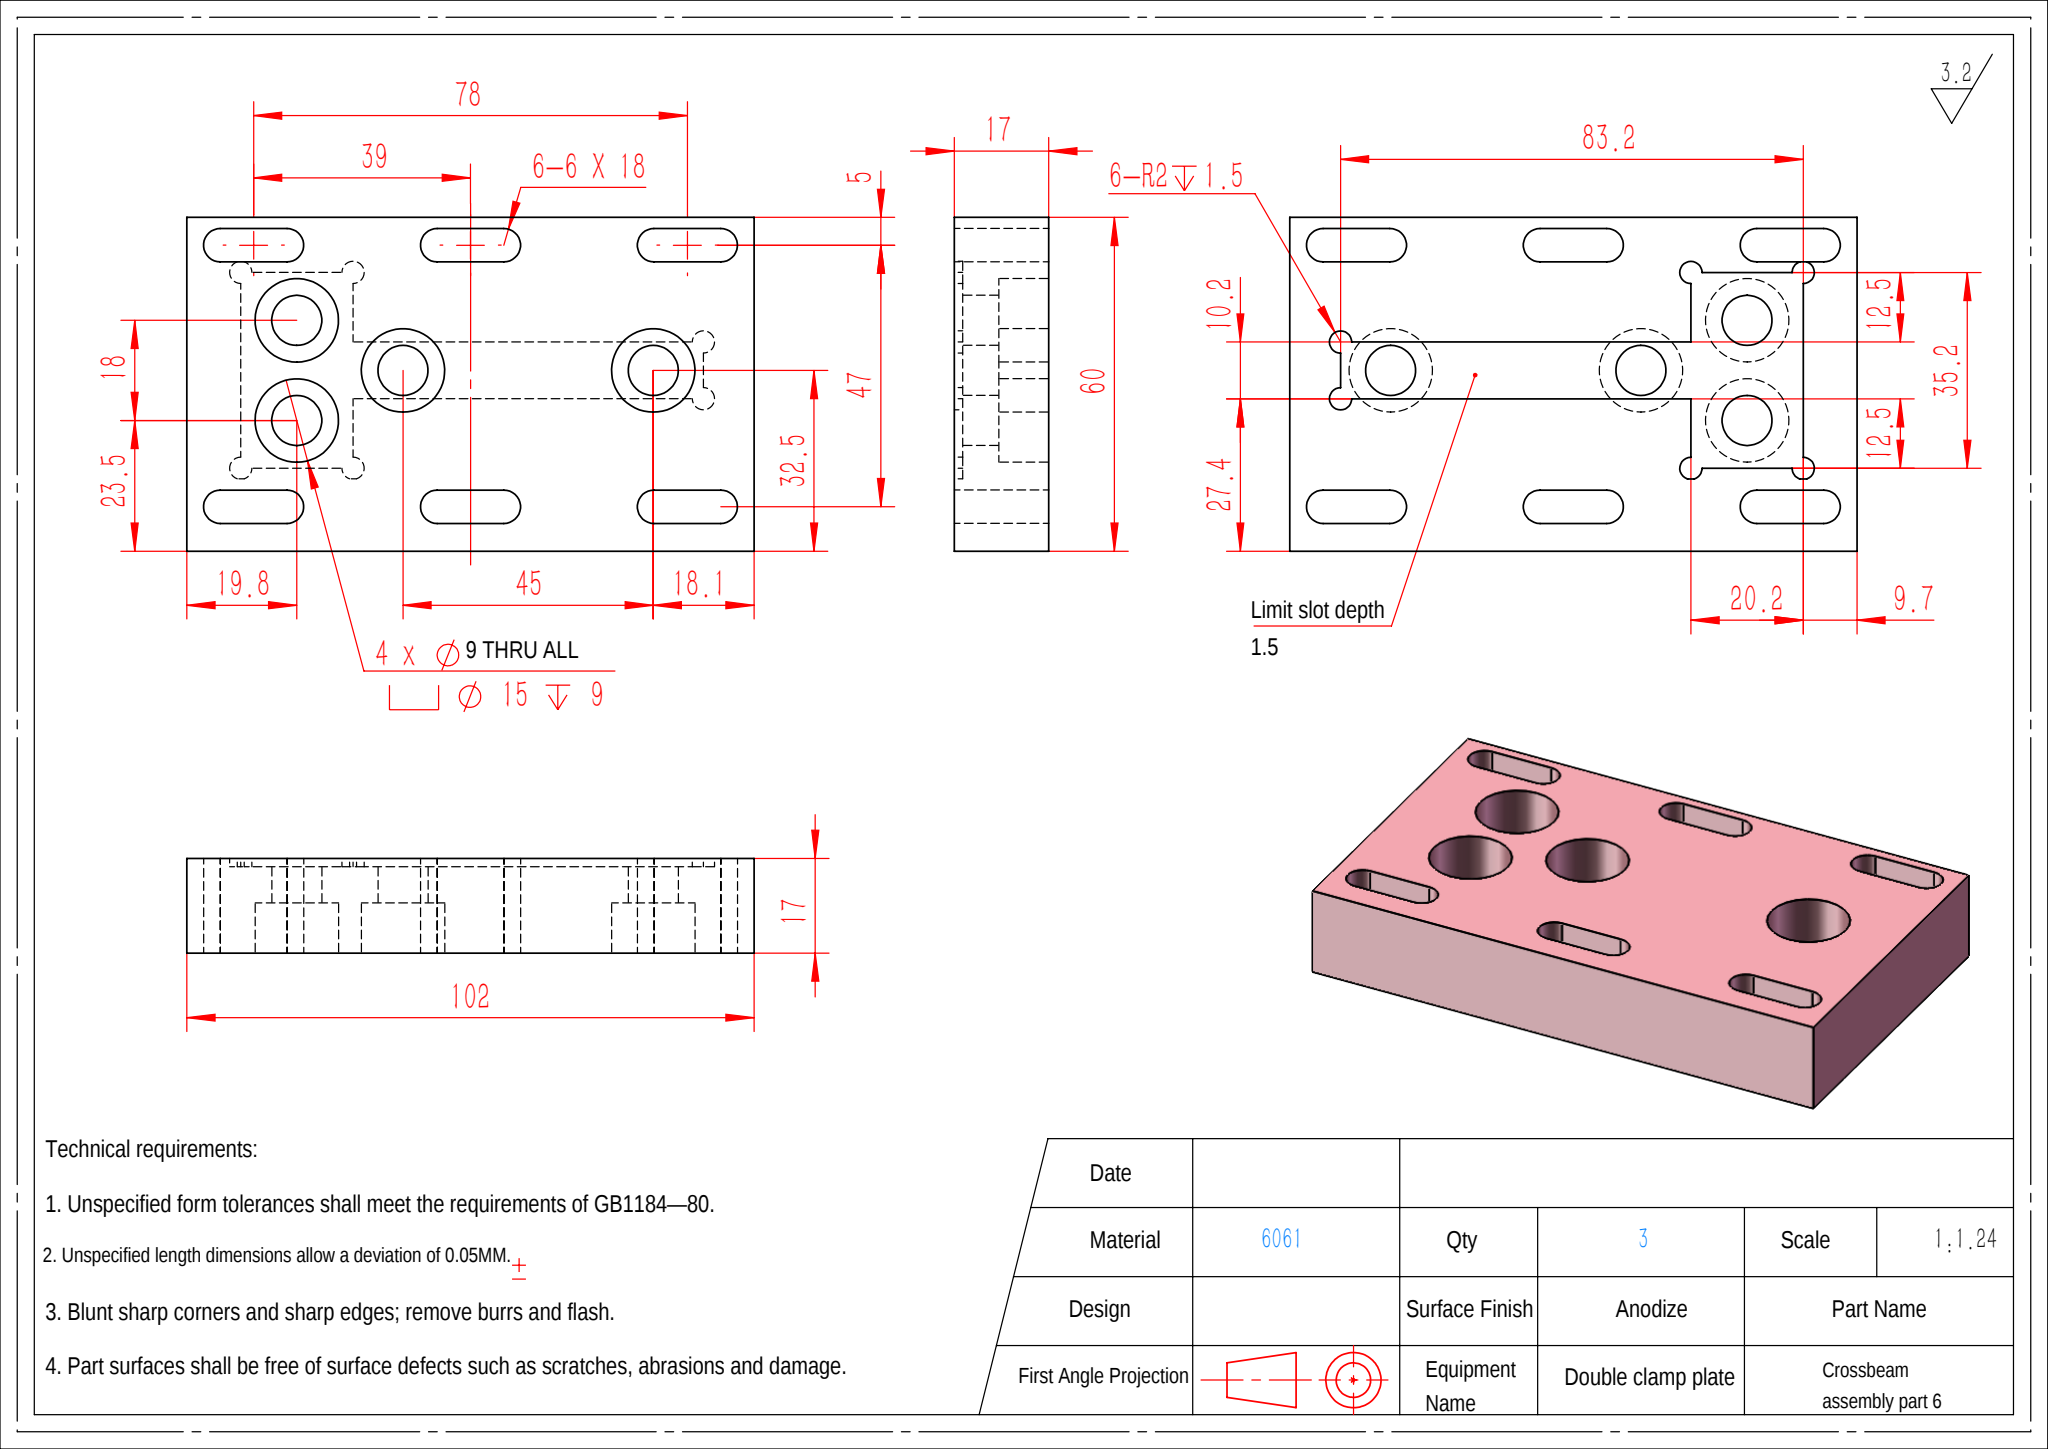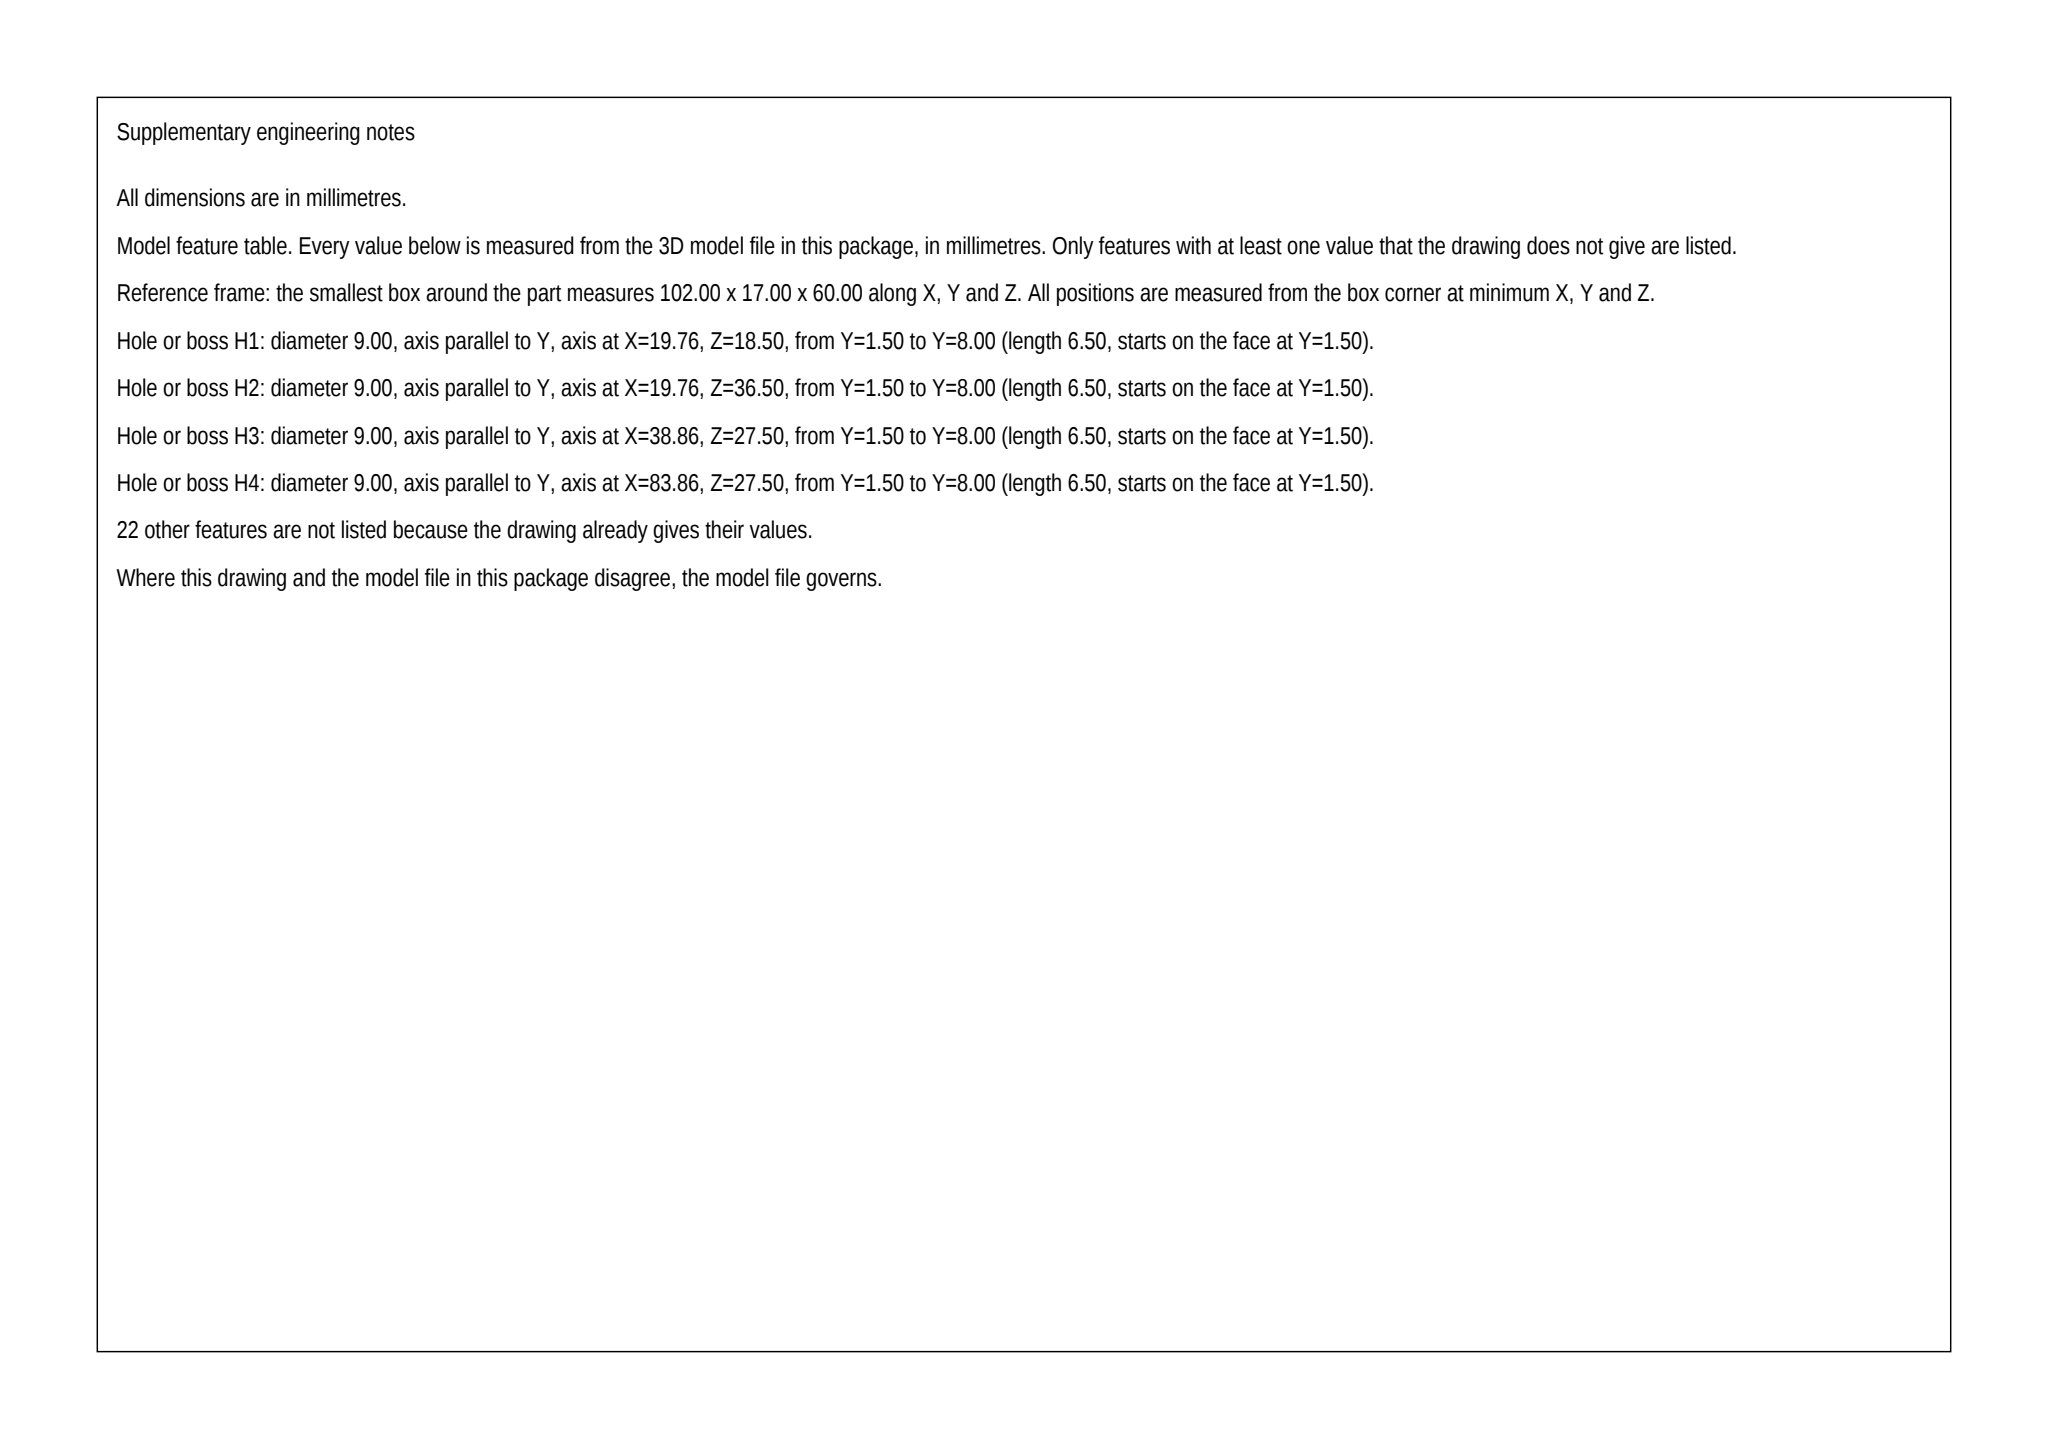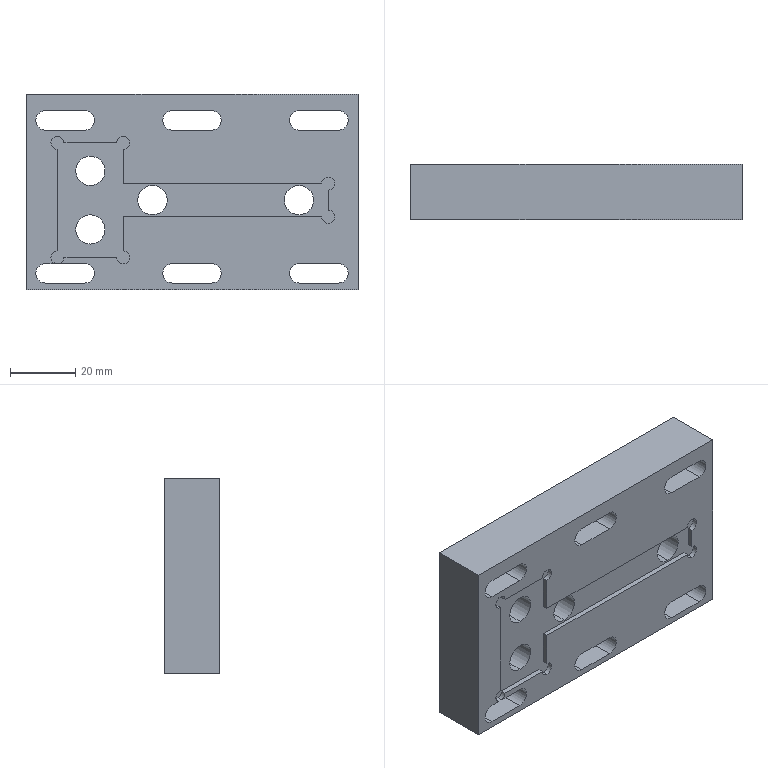Part | SolidWorks | mm | material 6061 | 1 solid | 72 faces | box 102 x 17 x 60 mm | volume 83681 mm3 | cylinder 39 | plane 33 | commonest cylinder face diameters 6 x12 4 x11 15 x8 9 x8
build123d program:
from build123d import *

# Parameters (mm, degrees)
SKETCH1_W                                           = 102
SKETCH1_H                                           = 60
BOSS_EXTRUDE1_DEPTH                                 = 8.5
CUT_EXTRUDE2_DEPTH                                  = 1.5
CUT_EXTRUDE4_DEPTH                                  = 62.563
CYLINDRICAL_COUNTERSUNK_HOLE_FOR_M8_HEX_D           = 9
CYLINDRICAL_COUNTERSUNK_HOLE_FOR_M8_HEX_DEPTH       = 17
CYLINDRICAL_COUNTERSUNK_HOLE_FOR_M8_HEX_CBORE_D     = 15
CYLINDRICAL_COUNTERSUNK_HOLE_FOR_M8_HEX_CBORE_DEPTH = 9
LPATTERN1_COUNT                                     = 2
LPATTERN1_PITCH                                     = 39
LPATTERN2_COPY_1_DEPTH                              = 62.563
LPATTERN2_COPY_2_DEPTH                              = 62.563
LPATTERN3_COUNT                                     = 2
LPATTERN3_PITCH                                     = 47
LPATTERN3_COPY_1_DEPTH                              = 62.563
LPATTERN3_COPY_2_DEPTH                              = 62.563
LPATTERN3_COPY_3_DEPTH                              = 62.563


with BuildPart() as part:
    # Sketch1 → Boss-Extrude1 (new, symmetric)
    with BuildSketch(Plane(origin=(0, 17, 0), x_dir=(1, 0, 0), z_dir=(0, 1, 0))):
        Rectangle(SKETCH1_W, SKETCH1_H)
    extrude(amount=BOSS_EXTRUDE1_DEPTH, both=True)

    # Sketch3 → Cut-Extrude2 (cut)
    with BuildSketch(Plane.XZ.offset(-8.5)):
        with BuildLine():
            Line((-39.336, -20.1), (-23.136, -20.1))
            ThreePointArc((-23.136, -20.1), (-19.722, -21.514), (-21.136, -18.1))
            Line((-21.136, -18.1), (-21.136, -7.6))
            Line((-21.136, -7.6), (39.864, -7.6))
            ThreePointArc((39.864, -7.6), (43.278, -9.014), (41.864, -5.6))
            Line((41.864, -5.6), (41.864, 0.6))
            ThreePointArc((41.864, 0.6), (43.278, 4.014), (39.864, 2.6))
            Line((39.864, 2.6), (-21.136, 2.6))
            Line((-21.136, 2.6), (-21.136, 13.1))
            ThreePointArc((-21.136, 13.1), (-19.161, 14.784), (-20.512, 17))
            Line((-20.512, 17), (-21.761, 17))
            ThreePointArc((-21.761, 17), (-22.756, 16.273), (-23.136, 15.1))
            Line((-23.136, 15.1), (-39.336, 15.1))
            ThreePointArc((-39.336, 15.1), (-39.716, 16.273), (-40.712, 17))
            Line((-40.712, 17), (-41.961, 17))
            ThreePointArc((-41.961, 17), (-43.311, 14.784), (-41.336, 13.1))
            Line((-41.336, 13.1), (-41.336, -18.1))
            ThreePointArc((-41.336, -18.1), (-43.311, -19.784), (-41.961, -22))
            Line((-41.961, -22), (-40.712, -22))
            ThreePointArc((-40.712, -22), (-39.716, -21.273), (-39.336, -20.1))
        make_face()
    extrude(amount=-CUT_EXTRUDE2_DEPTH, mode=Mode.SUBTRACT)

    # Sketch5 → Cut-Extrude4 (cut, through all)
    with BuildSketch(Plane(origin=(0, 25.5, 0), x_dir=(-1, 0, 0), z_dir=(0, 1, 0))):
        with BuildLine():
            Line((-6, 25), (6, 25))
            ThreePointArc((6, 25), (9, 22), (6, 19))
            Line((6, 19), (-6, 19))
            ThreePointArc((-6, 19), (-9, 22), (-6, 25))
        make_face()
    cut_extrude4 = extrude(amount=-CUT_EXTRUDE4_DEPTH, mode=Mode.SUBTRACT)

    # Cylindrical Countersunk Hole for M8 Hex
    with Locations(Plane(origin=(0, 25.5, 0), x_dir=(1, 0, 0), z_dir=(0, 1, 0))):
        with Locations((-31.236, 11.5), (-31.236, -6.5), (-12.136, 2.5), (32.864, 2.5)):
            CounterBoreHole(CYLINDRICAL_COUNTERSUNK_HOLE_FOR_M8_HEX_D / 2, CYLINDRICAL_COUNTERSUNK_HOLE_FOR_M8_HEX_CBORE_D / 2, CYLINDRICAL_COUNTERSUNK_HOLE_FOR_M8_HEX_CBORE_DEPTH, depth=CYLINDRICAL_COUNTERSUNK_HOLE_FOR_M8_HEX_DEPTH)

    # LPattern1: Cut-Extrude4 ×2
    with Locations(*[(-i * LPATTERN1_PITCH, 0, 0) for i in range(1, LPATTERN1_COUNT)]):
        add(cut_extrude4, mode=Mode.SUBTRACT)

    # LPattern2 copy 1 sketch → LPattern2 copy 1 (cut, through all)
    with BuildSketch(Plane(origin=(0, 25.5, 0), x_dir=(-1, 0, 0), z_dir=(0, 1, 0))):
        with BuildLine():
            Line((-6, 25), (6, 25))
            ThreePointArc((6, 25), (9, 22), (6, 19))
            Line((6, 19), (-6, 19))
            ThreePointArc((-6, 19), (-9, 22), (-6, 25))
        make_face()
    extrude(amount=-LPATTERN2_COPY_1_DEPTH, mode=Mode.SUBTRACT)

    # LPattern2 copy 2 sketch → LPattern2 copy 2 (cut, through all)
    with BuildSketch(Plane(origin=(39, 25.5, 0), x_dir=(-1, 0, 0), z_dir=(0, 1, 0))):
        with BuildLine():
            Line((-6, 25), (6, 25))
            ThreePointArc((6, 25), (9, 22), (6, 19))
            Line((6, 19), (-6, 19))
            ThreePointArc((-6, 19), (-9, 22), (-6, 25))
        make_face()
    extrude(amount=-LPATTERN2_COPY_2_DEPTH, mode=Mode.SUBTRACT)

    # LPattern3: Cut-Extrude4 ×2
    with Locations(*[(0, 0, -i * LPATTERN3_PITCH) for i in range(1, LPATTERN3_COUNT)]):
        add(cut_extrude4, mode=Mode.SUBTRACT)

    # LPattern3 copy 1 sketch → LPattern3 copy 1 (cut, through all)
    with BuildSketch(Plane(origin=(-39, 25.5, -47), x_dir=(-1, 0, 0), z_dir=(0, 1, 0))):
        with BuildLine():
            Line((-6, 25), (6, 25))
            ThreePointArc((6, 25), (9, 22), (6, 19))
            Line((6, 19), (-6, 19))
            ThreePointArc((-6, 19), (-9, 22), (-6, 25))
        make_face()
    extrude(amount=-LPATTERN3_COPY_1_DEPTH, mode=Mode.SUBTRACT)

    # LPattern3 copy 2 sketch → LPattern3 copy 2 (cut, through all)
    with BuildSketch(Plane(origin=(0, 25.5, -47), x_dir=(-1, 0, 0), z_dir=(0, 1, 0))):
        with BuildLine():
            Line((-6, 25), (6, 25))
            ThreePointArc((6, 25), (9, 22), (6, 19))
            Line((6, 19), (-6, 19))
            ThreePointArc((-6, 19), (-9, 22), (-6, 25))
        make_face()
    extrude(amount=-LPATTERN3_COPY_2_DEPTH, mode=Mode.SUBTRACT)

    # LPattern3 copy 3 sketch → LPattern3 copy 3 (cut, through all)
    with BuildSketch(Plane(origin=(39, 25.5, -47), x_dir=(-1, 0, 0), z_dir=(0, 1, 0))):
        with BuildLine():
            Line((-6, 25), (6, 25))
            ThreePointArc((6, 25), (9, 22), (6, 19))
            Line((6, 19), (-6, 19))
            ThreePointArc((-6, 19), (-9, 22), (-6, 25))
        make_face()
    extrude(amount=-LPATTERN3_COPY_3_DEPTH, mode=Mode.SUBTRACT)


solid = part.part